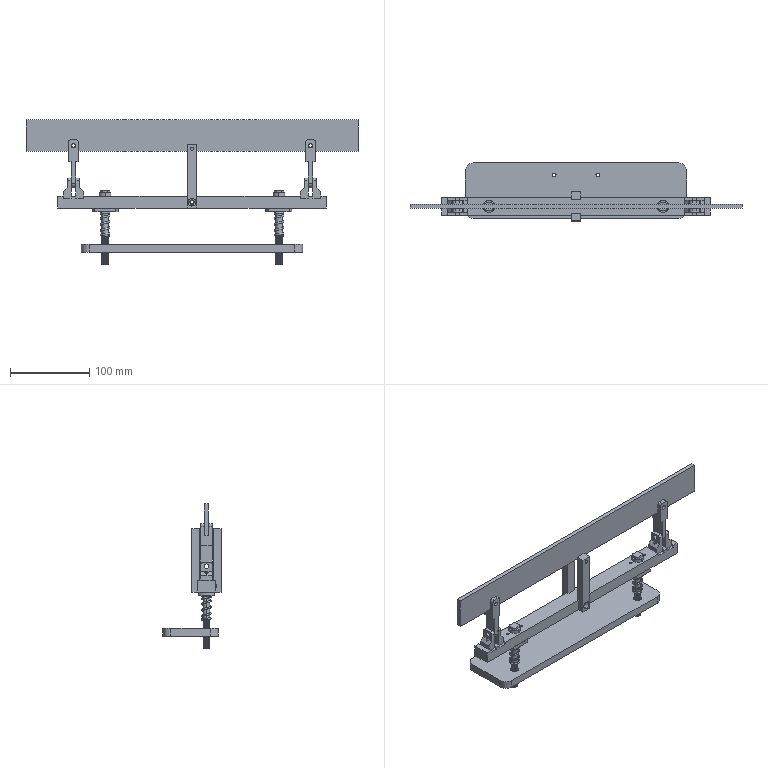Assembly | SolidWorks | mm | 17 component files | 17 solids | 427 faces | box 420 x 73.5 x 182.5 mm | volume 437904 mm3 | cylinder 258 | plane 155 | spline 10 | cone 4 | commonest cylinder face diameters 8 x132 6 x28 4.2 x22 10 x18 5.5 x14 4.5 x12 15 x8 3.3 x8
Bill of materials:
BeefTendon | 1 |  | Long, thin flat rectangular bar (strip) with two small round through holes, one near each end, both set off-center toward one long edge.
ConnectingHinge1 | 2 |  | Elongated link with a forked (slotted) wider end and a narrower tongue at the other end. The fork has rounded tops and a cross hole through both tines. The rounded tongue end has a through hole whose axis is perpendicular to the fork hole.
FixedRod | 1 |  | Long rectangular-section bar, symmetric about its center. Near each end the top face has two shallow transverse grooves, two small holes, and one large round bore flanked by two small holes. At mid-length both sides are notched to a narrower width, and a small horizontal cross hole runs through the side face.
GuideRod | 2 |  | Headed bolt or pin: a short head that is round with two parallel flats, a long plain cylindrical shank, and helical thread geometry over roughly the last third of the length toward the tip.
LeftLocatingPlate | 1 |  | Square-section prismatic bar with two transverse through holes on the same face, one near each end. The hole near one end is noticeably larger than the hole near the other.
LinearBearing8uu | 2 |  | Flanged bushing or boss: a cylindrical sleeve with a central through bore standing on a flat flange. The flange has two parallel straight sides and two convex arc ends, with one mounting hole near each arc end.
RightLocatingPlate | 1 |  | Square-section prismatic bar with two equal-size transverse through holes on one face, one near each end.
Spring | 2 | 45 | Helical coil spring made of round wire, with about 6 open coils at roughly uniform pitch and cut wire ends.
TelescopicCylinderFixedLead-outPlate | 1 |  | Flat rectangular plate with rounded corners. Two larger holes sit near the ends along one long edge, and two smaller holes sit closer to the middle near the opposite long edge.
UpperHinge | 4 |  | Block-shaped bracket or lug. The upper portion is thinner, with a rounded top and a large through hole. The lower portion is thicker and connects to the upper portion through an inclined (chamfer-like) face. A smaller hole opens on the inclined face.
Mates:
1. concentric | FixedRod-1 face at (140, -208.228, 63.5) dir (0, -1, 0) r 2.5 | RightLocatingPlate-1 face at (140, -200.728, 63.5) dir (0, 1, 0) r 2.1
2. coincident | FixedRod-1 face at (-30, -210.728, 56) dir (0, 1, 0) | RightLocatingPlate-1 face at (146, -210.728, 136) dir (0, -1, 0)
3. coincident | FixedRod-1 face at (146, -210.728, 71) dir (-1, 0, 0) | RightLocatingPlate-1 face at (146, -200.728, 136) dir (1, 0, 0)
4. concentric | FixedRod-1 face at (30, -219.228, 56) dir (0, 0, -1) r 7.5 | LinearBearing8uu-1 face at (30, -219.228, 26.839) dir (0, 0, -1) r 7.5
5. coincident | FixedRod-1 face at (-30, -230.228, 56) dir (0, 0, -1) | LinearBearing8uu-1 face at (13.5, -219.228, 56) dir (0, 0, 1)
6. parallel | FixedRod-1 face at (-30, -230.228, 71) dir (0, -1, 0) | LinearBearing8uu-1 face at (12.289, -229.728, 61) dir (0, -1, 0)
7. concentric | FixedRod-1 face at (-2, -219.228, 56) dir (0, 0, -1) r 5 | UpperHinge-1 face at (-2, -219.228, 68.5) dir (0, 0, -1) r 2.1
8. coincident | FixedRod-1 face at (-30, -230.228, 68.5) dir (0, 0, 1) | UpperHinge-1 face at (3, -211.728, 68.5) dir (0, 0, -1)
9. parallel | FixedRod-1 face at (-30, -208.228, 71) dir (0, 1, 0) | UpperHinge-1 face at (3, -211.728, 93.5) dir (0, 1, 0)
10. coincident | FixedRod-1 face at (-30, -230.228, 68.5) dir (0, 0, 1) | UpperHinge-2 face at (-23, -226.728, 68.5) dir (0, 0, -1)
11. concentric | FixedRod-1 face at (-18, -219.228, 56) dir (0, 0, -1) r 5 | UpperHinge-2 face at (-18, -219.228, 68.5) dir (0, 0, -1) r 2.1
12. coincident | FixedRod-1 face at (-23, -208.228, 68.5) dir (1, 0, 0) | UpperHinge-2 face at (-23, -226.728, 93.5) dir (-1, 0, 0)
13. concentric | ConnectingHinge1-2 face at (-4, -219.228, 88.5) dir (-1, 0, 0) r 3 | UpperHinge-2 face at (-13, -219.228, 88.5) dir (-1, 0, 0) r 3
14. coincident | ConnectingHinge1-2 face at (-13, -226.728, 82.5) dir (-1, 0, 0) | UpperHinge-2 face at (-13, -226.728, 93.5) dir (1, 0, 0)
15. concentric | ConnectingHinge1-1 face at (290, -211.727, 135) dir (0, -1, 0) r 2.75 | BeefTendon-1 face at (290, -216.728, 135) dir (0, 1, 0) r 2.1
16. concentric | ConnectingHinge1-2 face at (-10, -211.727, 135) dir (0, -1, 0) r 2.75 | BeefTendon-1 face at (-10, -216.728, 135) dir (0, 1, 0) r 2.1
17. coincident | ConnectingHinge1-2 face at (-16, -216.728, 127.5) dir (0, -1, 0) | BeefTendon-1 face at (-70, -216.728, 167.5) dir (0, 1, 0)
18. concentric | ConnectingHinge1-1 face at (296, -219.228, 88.5) dir (-1, 0, 0) r 3 | UpperHinge-4 face at (287, -219.228, 88.5) dir (-1, 0, 0) r 3
19. coincident | ConnectingHinge1-1 face at (287, -226.728, 82.5) dir (-1, 0, 0) | UpperHinge-4 face at (287, -226.728, 93.5) dir (1, 0, 0)
20. concentric | ConnectingHinge1-1 face at (296, -219.228, 88.5) dir (-1, 0, 0) r 3 | UpperHinge-4 face at (287, -219.228, 88.5) dir (-1, 0, 0) r 3
21. concentric | UpperHinge-3 face at (298, -219.228, 68.5) dir (0, 0, -1) r 2.1 | FixedRod-1 face at (298, -219.228, 56) dir (0, 0, -1) r 2.75
22. coincident | UpperHinge-3 face at (303, -211.728, 68.5) dir (0, 0, -1) | FixedRod-1 face at (-30, -230.228, 68.5) dir (0, 0, 1)
23. concentric | UpperHinge-4 face at (282, -219.228, 68.5) dir (0, 0, -1) r 2.1 | FixedRod-1 face at (282, -219.228, 56) dir (0, 0, -1) r 2.75
24. coincident | UpperHinge-4 face at (277, -226.728, 68.5) dir (0, 0, -1) | FixedRod-1 face at (-30, -230.228, 68.5) dir (0, 0, 1)
25. concentric | FixedRod-1 face at (140, -208.228, 63.5) dir (0, -1, 0) r 2.5 | LeftLocatingPlate-1 face at (140, -237.728, 63.5) dir (0, -1, 0) r 5
26. coincident | FixedRod-1 face at (-30, -227.728, 56) dir (0, -1, 0) | LeftLocatingPlate-1 face at (134, -227.728, 136) dir (0, 1, 0)
27. parallel | FixedRod-1 face at (-30, -208.228, 71) dir (0, 1, 0) | GuideRod-1 face at (246.683, -214.228, -15) dir (0, 1, 0)
28. coincident | FixedRod-1 face at (146, -227.728, 71) dir (-1, 0, 0) | LeftLocatingPlate-1 face at (146, -237.728, 136) dir (1, 0, 0)
29. concentric | TelescopicCylinderFixedLead-outPlate-1 face at (250, -219.228, 0) dir (0, 0, 1) r 5 | GuideRod-1 face at (250, -219.228, -15) dir (0, 0, 1) r 4
30. distance | GuideRod-1 face at (250, -219.228, -15) dir (0, 0, -1) | TelescopicCylinderFixedLead-outPlate-1 face at (280, -164.228, 0) dir (0, 0, -1)
31. concentric | TelescopicCylinderFixedLead-outPlate-1 face at (30, -219.228, 0) dir (0, 0, 1) r 5 | GuideRod-2 face at (30, -219.228, -15) dir (0, 0, 1) r 4
32. concentric | GuideRod-1 face at (250, -219.228, -15) dir (0, 0, 1) r 4 | Spring-1 sketch segment at (250, -219.228, 51) dir (0, 0, -1) r 5.2
33. coincident | GuideRod-1 face at (250, -219.228, -15) dir (0, 0, -1) | GuideRod-2 face at (30, -219.228, -15) dir (0, 0, -1)
34. coincident | TelescopicCylinderFixedLead-outPlate-1 face at (280, -164.228, 0) dir (0, 0, -1) | assembly plane at (0, 0, 0) dir (0, 0, 1)
35. coincident | TelescopicCylinderFixedLead-outPlate-1 face at (0, -164.228, 10) dir (-1, 0, 0) | assembly plane at (0, 0, 0) dir (1, 0, 0)
36. concentric | LinearBearing8uu-1 face at (30, -219.228, 26.839) dir (0, 0, -1) r 4 | GuideRod-2 face at (30, -219.228, -15) dir (0, 0, 1) r 4
37. coincident | LinearBearing8uu-1 face at (22.5, -219.228, 75) dir (0, 0, 1) | GuideRod-2 face at (30, -219.228, 75) dir (0, 0, -1)
38. parallel | TelescopicCylinderFixedLead-outPlate-1 face at (280, -234.228, 10) dir (0, -1, 0) | GuideRod-2 face at (33.317, -224.228, -15) dir (0, -1, 0)
39. concentric | FixedRod-1 face at (250, -219.228, 56) dir (0, 0, -1) r 7.5 | LinearBearing8uu-2 face at (250, -219.228, 26.839) dir (0, 0, -1) r 7.5
40. coincident | FixedRod-1 face at (-30, -230.228, 56) dir (0, 0, -1) | LinearBearing8uu-2 face at (233.5, -219.228, 56) dir (0, 0, 1)
41. concentric | GuideRod-1 face at (250, -219.228, -15) dir (0, 0, 1) r 4 | LinearBearing8uu-2 face at (250, -219.228, 26.839) dir (0, 0, -1) r 4
42. coincident | Spring-1 sketch segment at (250, -219.228, 51) dir (0, 0, -1) r 5.2 | LinearBearing8uu-2 face at (246, -219.228, 51) dir (0, 0, -1)
43. parallel | BeefTendon-1 face at (-70, -216.728, 127.5) dir (0, 0, -1) | FixedRod-1 face at (-30, -230.228, 56) dir (0, 0, -1)
44. concentric | GuideRod-2 face at (30, -219.228, -15) dir (0, 0, 1) r 4 | Spring-2 sketch segment at (30, -219.228, 51) dir (0, 0, -1) r 5.2
45. coincident | LinearBearing8uu-1 face at (26, -219.228, 51) dir (0, 0, -1) | Spring-2 face at (30, -219.228, 51) dir (0, 0, 1)
46. concentric | FixedRod-1 face at (238, -219.228, 71) dir (0, 0, 1) r 1.65 | LinearBearing8uu-2 face at (238, -219.228, 51) dir (0, 0, -1) r 4